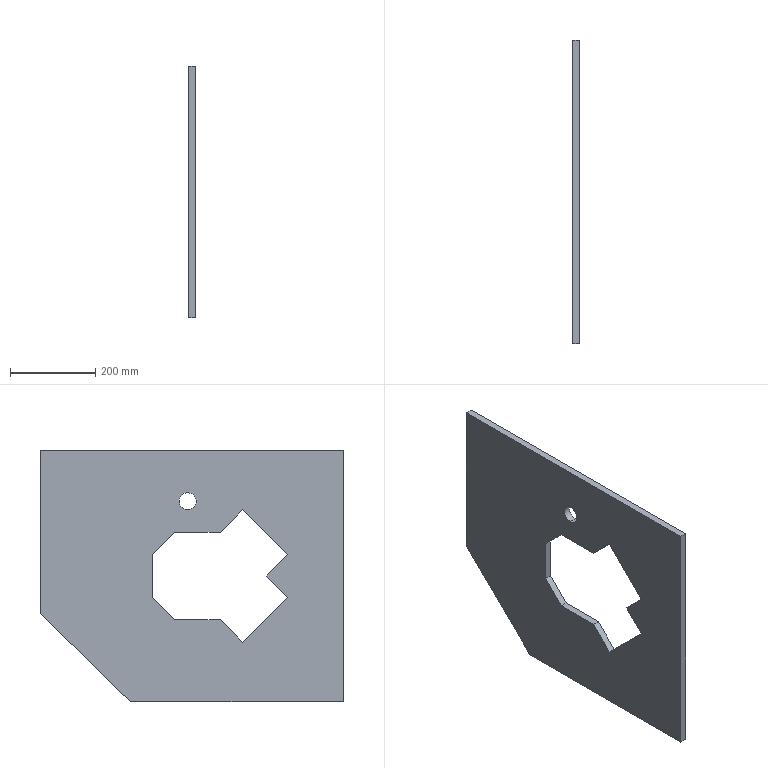Component | SolidWorks | AssemblyDriveAxis-1_16PlateModified-1 | 1 solid | 25 faces | box 16 x 710 x 590 mm | volume 5329547 mm3 | plane 23 | cylinder 2 | commonest cylinder face diameters 40 x2
build123d program:
from build123d import *

# Parameters (mm, degrees)
SKETCH1_2_W          = 590
SKETCH1_2_H          = 710
BOSS_EXTRUDE1_DEPTH  = 16
SKETCH2_R            = 20
CUT_EXTRUDE1_2_DEPTH = 16
CUT_EXTRUDE3_DEPTH   = 16
CUT_EXTRUDE1_DEPTH   = 3.5


with BuildPart() as part:
    # Sketch1_2 → Boss-Extrude1 (new body)
    with BuildSketch(Plane.XY):
        with Locations((295, 355)):
            Rectangle(SKETCH1_2_W, SKETCH1_2_H)
    extrude(amount=BOSS_EXTRUDE1_DEPTH)

    # Sketch2 → Cut-Extrude1_2 (cut)
    with BuildSketch(Plane.XY.offset(16)):
        Polygon((345, 448), (245, 448), (193, 396), (193, 289), (140, 236), (245.738, 130.262), (295, 179.524), (344.262, 130.262), (450, 236), (397, 289), (397, 396), align=None)
        with Locations((120, 365)):
            Circle(SKETCH2_R)
    extrude(amount=-CUT_EXTRUDE1_2_DEPTH, mode=Mode.SUBTRACT)

    # Sketch4 → Cut-Extrude3 (cut)
    with BuildSketch(Plane.XY.offset(16)):
        Polygon((590, 498.948), (383.169, 710), (590, 710), align=None)
    extrude(amount=-CUT_EXTRUDE3_DEPTH, mode=Mode.SUBTRACT)

    # Sketch1 → Cut-Extrude1 (cut)
    with BuildSketch(Plane.XY.offset(16)):
        Polygon((337.078, 75.224), (314.451, 97.852), (334.25, 117.651), (356.877, 95.023), align=None)
    extrude(amount=-CUT_EXTRUDE1_DEPTH, mode=Mode.SUBTRACT)


solid = part.part

# Placed as in the assembly
solid = solid.moved(Location((-141, 500, 565), (0, 90, 0)))
STEP:
#1=CARTESIAN_POINT('',(-5.551,34.055,18.307));
#2=VERTEX_POINT('',#1);
#3=CARTESIAN_POINT('',(-5.551,34.055,16.732));
#4=VERTEX_POINT('',#3);
#5=CARTESIAN_POINT('',(-5.551,34.055,17.52));
#6=DIRECTION('',(1.,-0.,0.));
#7=DIRECTION('',(0.,0.,-1.));
#8=AXIS2_PLACEMENT_3D('',#5,#6,#7);
#9=CIRCLE('',#8,0.7874);
#10=EDGE_CURVE('',#2,#4,#9,.T.);
#11=ORIENTED_EDGE('',*,*,#10,.F.);
#12=CARTESIAN_POINT('',(-4.921,34.055,18.307));
#13=VERTEX_POINT('',#12);
#14=CARTESIAN_POINT('',(-5.551,34.055,18.307));
#15=DIRECTION('',(1.,-0.,0.));
#16=VECTOR('',#15,39.37);
#17=LINE('',#14,#16);
#18=EDGE_CURVE('',#2,#13,#17,.T.);
#19=ORIENTED_EDGE('',*,*,#18,.T.);
#20=CARTESIAN_POINT('',(-4.921,34.055,16.732));
#21=VERTEX_POINT('',#20);
#22=CARTESIAN_POINT('',(-4.921,34.055,17.52));
#23=DIRECTION('',(1.,-0.,0.));
#24=DIRECTION('',(0.,0.,-1.));
#25=AXIS2_PLACEMENT_3D('',#22,#23,#24);
#26=CIRCLE('',#25,0.7874);
#27=EDGE_CURVE('',#13,#21,#26,.T.);
#28=ORIENTED_EDGE('',*,*,#27,.T.);
#29=CARTESIAN_POINT('',(-5.551,34.055,16.732));
#30=DIRECTION('',(1.,-0.,0.));
#31=VECTOR('',#30,39.37);
#32=LINE('',#29,#31);
#33=EDGE_CURVE('',#4,#21,#32,.T.);
#34=ORIENTED_EDGE('',*,*,#33,.F.);
#35=EDGE_LOOP('',(#11,#19,#28,#34));
#36=FACE_OUTER_BOUND('',#35,.T.);
#37=CARTESIAN_POINT('',(-5.551,34.055,17.52));
#38=DIRECTION('',(1.,-0.,0.));
#39=DIRECTION('',(0.,0.,-1.));
#40=AXIS2_PLACEMENT_3D('',#37,#38,#39);
#41=CYLINDRICAL_SURFACE('',#40,0.7874);
#42=ADVANCED_FACE('',(#36),#41,.F.);
#43=CARTESIAN_POINT('',(-4.921,22.647,8.973));
#44=VERTEX_POINT('',#43);
#45=CARTESIAN_POINT('',(-4.921,23.426,8.194));
#46=VERTEX_POINT('',#45);
#47=CARTESIAN_POINT('',(-4.921,23.426,8.194));
#48=DIRECTION('',(0.,0.7071,-0.7071));
#49=VECTOR('',#48,39.37);
#50=LINE('',#47,#49);
#51=EDGE_CURVE('',#44,#46,#50,.T.);
#52=ORIENTED_EDGE('',*,*,#51,.F.);
#53=CARTESIAN_POINT('',(-4.921,23.537,9.864));
#54=VERTEX_POINT('',#53);
#55=CARTESIAN_POINT('',(-4.921,22.647,8.973));
#56=DIRECTION('',(-0.,-0.7071,-0.7071));
#57=VECTOR('',#56,39.37);
#58=LINE('',#55,#57);
#59=EDGE_CURVE('',#54,#44,#58,.T.);
#60=ORIENTED_EDGE('',*,*,#59,.F.);
#61=CARTESIAN_POINT('',(-4.921,24.317,9.085));
#62=VERTEX_POINT('',#61);
#63=CARTESIAN_POINT('',(-4.921,23.537,9.864));
#64=DIRECTION('',(-0.,-0.7071,0.7071));
#65=VECTOR('',#64,39.37);
#66=LINE('',#63,#65);
#67=EDGE_CURVE('',#62,#54,#66,.T.);
#68=ORIENTED_EDGE('',*,*,#67,.F.);
#69=CARTESIAN_POINT('',(-4.921,24.317,9.085));
#70=DIRECTION('',(0.,0.7071,0.7071));
#71=VECTOR('',#70,39.37);
#72=LINE('',#69,#71);
#73=EDGE_CURVE('',#46,#62,#72,.T.);
#74=ORIENTED_EDGE('',*,*,#73,.F.);
#75=EDGE_LOOP('',(#52,#60,#68,#74));
#76=FACE_BOUND('',#75,.T.);
#77=CARTESIAN_POINT('',(-4.921,47.638,7.159));
#78=VERTEX_POINT('',#77);
#79=CARTESIAN_POINT('',(-4.921,39.329,-0.9843));
#80=VERTEX_POINT('',#79);
#81=CARTESIAN_POINT('',(-4.921,39.329,-0.9843));
#82=DIRECTION('',(-0.,-0.7142,-0.6999));
#83=VECTOR('',#82,39.37);
#84=LINE('',#81,#83);
#85=EDGE_CURVE('',#78,#80,#84,.T.);
#86=ORIENTED_EDGE('',*,*,#85,.F.);
#87=CARTESIAN_POINT('',(-4.921,47.638,22.244));
#88=VERTEX_POINT('',#87);
#89=CARTESIAN_POINT('',(-4.921,47.638,-0.9843));
#90=DIRECTION('',(-0.,0.,1.));
#91=VECTOR('',#90,39.37);
#92=LINE('',#89,#91);
#93=EDGE_CURVE('',#78,#88,#92,.T.);
#94=ORIENTED_EDGE('',*,*,#93,.T.);
#95=CARTESIAN_POINT('',(-4.921,19.685,22.244));
#96=VERTEX_POINT('',#95);
#97=CARTESIAN_POINT('',(-4.921,47.638,22.244));
#98=DIRECTION('',(-0.,-1.,-0.));
#99=VECTOR('',#98,39.37);
#100=LINE('',#97,#99);
#101=EDGE_CURVE('',#88,#96,#100,.T.);
#102=ORIENTED_EDGE('',*,*,#101,.T.);
#103=CARTESIAN_POINT('',(-4.921,19.685,-0.9843));
#104=VERTEX_POINT('',#103);
#105=CARTESIAN_POINT('',(-4.921,19.685,22.244));
#106=DIRECTION('',(0.,0.,-1.));
#107=VECTOR('',#106,39.37);
#108=LINE('',#105,#107);
#109=EDGE_CURVE('',#96,#104,#108,.T.);
#110=ORIENTED_EDGE('',*,*,#109,.T.);
#111=CARTESIAN_POINT('',(-4.921,19.685,-0.9843));
#112=DIRECTION('',(0.,1.,0.));
#113=VECTOR('',#112,39.37);
#114=LINE('',#111,#113);
#115=EDGE_CURVE('',#104,#80,#114,.T.);
#116=ORIENTED_EDGE('',*,*,#115,.T.);
#117=EDGE_LOOP('',(#86,#94,#102,#110,#116));
#118=FACE_OUTER_BOUND('',#117,.T.);
#119=CARTESIAN_POINT('',(-4.921,34.055,17.52));
#120=DIRECTION('',(1.,-0.,0.));
#121=DIRECTION('',(0.,0.,-1.));
#122=AXIS2_PLACEMENT_3D('',#119,#120,#121);
#123=CIRCLE('',#122,0.7874);
#124=EDGE_CURVE('',#21,#13,#123,.T.);
#125=ORIENTED_EDGE('',*,*,#124,.F.);
#126=ORIENTED_EDGE('',*,*,#27,.F.);
#127=EDGE_LOOP('',(#125,#126));
#128=FACE_BOUND('',#127,.T.);
#129=CARTESIAN_POINT('',(-4.921,37.323,12.598));
#130=VERTEX_POINT('',#129);
#131=CARTESIAN_POINT('',(-4.921,35.276,14.646));
#132=VERTEX_POINT('',#131);
#133=CARTESIAN_POINT('',(-4.921,23.681,26.24));
#134=DIRECTION('',(-0.,-0.7071,0.7071));
#135=VECTOR('',#134,39.37);
#136=LINE('',#133,#135);
#137=EDGE_CURVE('',#130,#132,#136,.T.);
#138=ORIENTED_EDGE('',*,*,#137,.F.);
#139=CARTESIAN_POINT('',(-4.921,37.323,8.661));
#140=VERTEX_POINT('',#139);
#141=CARTESIAN_POINT('',(-4.921,37.323,22.244));
#142=DIRECTION('',(0.,0.,-1.));
#143=VECTOR('',#142,39.37);
#144=LINE('',#141,#143);
#145=EDGE_CURVE('',#130,#140,#144,.T.);
#146=ORIENTED_EDGE('',*,*,#145,.T.);
#147=CARTESIAN_POINT('',(-4.921,35.276,6.614));
#148=VERTEX_POINT('',#147);
#149=CARTESIAN_POINT('',(-4.921,35.295,6.634));
#150=DIRECTION('',(-0.,-0.7071,-0.7071));
#151=VECTOR('',#150,39.37);
#152=LINE('',#149,#151);
#153=EDGE_CURVE('',#140,#148,#152,.T.);
#154=ORIENTED_EDGE('',*,*,#153,.T.);
#155=CARTESIAN_POINT('',(-4.921,31.063,6.614));
#156=VERTEX_POINT('',#155);
#157=CARTESIAN_POINT('',(-4.921,19.685,6.614));
#158=DIRECTION('',(-0.,-1.,0.));
#159=VECTOR('',#158,39.37);
#160=LINE('',#157,#159);
#161=EDGE_CURVE('',#148,#156,#160,.T.);
#162=ORIENTED_EDGE('',*,*,#161,.T.);
#163=CARTESIAN_POINT('',(-4.921,28.976,4.528));
#164=VERTEX_POINT('',#163);
#165=CARTESIAN_POINT('',(-4.921,33.189,8.74));
#166=DIRECTION('',(-0.,-0.7071,-0.7071));
#167=VECTOR('',#166,39.37);
#168=LINE('',#165,#167);
#169=EDGE_CURVE('',#156,#164,#168,.T.);
#170=ORIENTED_EDGE('',*,*,#169,.T.);
#171=CARTESIAN_POINT('',(-4.921,24.813,8.69));
#172=VERTEX_POINT('',#171);
#173=CARTESIAN_POINT('',(-4.921,15.472,18.031));
#174=DIRECTION('',(-0.,-0.7071,0.7071));
#175=VECTOR('',#174,39.37);
#176=LINE('',#173,#175);
#177=EDGE_CURVE('',#164,#172,#176,.T.);
#178=ORIENTED_EDGE('',*,*,#177,.T.);
#179=CARTESIAN_POINT('',(-4.921,26.753,10.63));
#180=VERTEX_POINT('',#179);
#181=CARTESIAN_POINT('',(-4.921,29.026,12.903));
#182=DIRECTION('',(0.,0.7071,0.7071));
#183=VECTOR('',#182,39.37);
#184=LINE('',#181,#183);
#185=EDGE_CURVE('',#172,#180,#184,.T.);
#186=ORIENTED_EDGE('',*,*,#185,.T.);
#187=CARTESIAN_POINT('',(-4.921,24.813,12.569));
#188=VERTEX_POINT('',#187);
#189=CARTESIAN_POINT('',(-4.921,17.412,19.971));
#190=DIRECTION('',(0.,0.7071,-0.7071));
#191=VECTOR('',#190,39.37);
#192=LINE('',#189,#191);
#193=EDGE_CURVE('',#188,#180,#192,.T.);
#194=ORIENTED_EDGE('',*,*,#193,.F.);
#195=CARTESIAN_POINT('',(-4.921,28.976,16.732));
#196=VERTEX_POINT('',#195);
#197=CARTESIAN_POINT('',(-4.921,27.087,14.843));
#198=DIRECTION('',(-0.,-0.7071,-0.7071));
#199=VECTOR('',#198,39.37);
#200=LINE('',#197,#199);
#201=EDGE_CURVE('',#196,#188,#200,.T.);
#202=ORIENTED_EDGE('',*,*,#201,.F.);
#203=CARTESIAN_POINT('',(-4.921,31.063,14.646));
#204=VERTEX_POINT('',#203);
#205=CARTESIAN_POINT('',(-4.921,21.575,24.134));
#206=DIRECTION('',(-0.,-0.7071,0.7071));
#207=VECTOR('',#206,39.37);
#208=LINE('',#205,#207);
#209=EDGE_CURVE('',#204,#196,#208,.T.);
#210=ORIENTED_EDGE('',*,*,#209,.F.);
#211=CARTESIAN_POINT('',(-4.921,19.685,14.646));
#212=DIRECTION('',(-0.,-1.,-0.));
#213=VECTOR('',#212,39.37);
#214=LINE('',#211,#213);
#215=EDGE_CURVE('',#132,#204,#214,.T.);
#216=ORIENTED_EDGE('',*,*,#215,.F.);
#217=EDGE_LOOP('',(#138,#146,#154,#162,#170,#178,#186,#194,#202,#210,#216));
#218=FACE_BOUND('',#217,.T.);
#219=CARTESIAN_POINT('',(-4.921,19.685,22.244));
#220=DIRECTION('',(1.,-0.,0.));
#221=DIRECTION('',(0.,0.,-1.));
#222=AXIS2_PLACEMENT_3D('',#219,#220,#221);
#223=PLANE('',#222);
#224=ADVANCED_FACE('',(#76,#118,#128,#218),#223,.T.);
#225=CARTESIAN_POINT('',(-5.551,34.055,17.52));
#226=DIRECTION('',(1.,-0.,0.));
#227=DIRECTION('',(0.,0.,-1.));
#228=AXIS2_PLACEMENT_3D('',#225,#226,#227);
#229=CIRCLE('',#228,0.7874);
#230=EDGE_CURVE('',#4,#2,#229,.T.);
#231=ORIENTED_EDGE('',*,*,#230,.T.);
#232=ORIENTED_EDGE('',*,*,#10,.T.);
#233=EDGE_LOOP('',(#231,#232));
#234=FACE_BOUND('',#233,.T.);
#235=CARTESIAN_POINT('',(-5.551,47.638,7.159));
#236=VERTEX_POINT('',#235);
#237=CARTESIAN_POINT('',(-5.551,47.638,22.244));
#238=VERTEX_POINT('',#237);
#239=CARTESIAN_POINT('',(-5.551,47.638,-0.9843));
#240=DIRECTION('',(-0.,0.,1.));
#241=VECTOR('',#240,39.37);
#242=LINE('',#239,#241);
#243=EDGE_CURVE('',#236,#238,#242,.T.);
#244=ORIENTED_EDGE('',*,*,#243,.F.);
#245=CARTESIAN_POINT('',(-5.551,39.329,-0.9843));
#246=VERTEX_POINT('',#245);
#247=CARTESIAN_POINT('',(-5.551,39.329,-0.9843));
#248=DIRECTION('',(-0.,-0.7142,-0.6999));
#249=VECTOR('',#248,39.37);
#250=LINE('',#247,#249);
#251=EDGE_CURVE('',#236,#246,#250,.T.);
#252=ORIENTED_EDGE('',*,*,#251,.T.);
#253=CARTESIAN_POINT('',(-5.551,19.685,-0.9843));
#254=VERTEX_POINT('',#253);
#255=CARTESIAN_POINT('',(-5.551,19.685,-0.9843));
#256=DIRECTION('',(0.,1.,0.));
#257=VECTOR('',#256,39.37);
#258=LINE('',#255,#257);
#259=EDGE_CURVE('',#254,#246,#258,.T.);
#260=ORIENTED_EDGE('',*,*,#259,.F.);
#261=CARTESIAN_POINT('',(-5.551,19.685,22.244));
#262=VERTEX_POINT('',#261);
#263=CARTESIAN_POINT('',(-5.551,19.685,22.244));
#264=DIRECTION('',(0.,0.,-1.));
#265=VECTOR('',#264,39.37);
#266=LINE('',#263,#265);
#267=EDGE_CURVE('',#262,#254,#266,.T.);
#268=ORIENTED_EDGE('',*,*,#267,.F.);
#269=CARTESIAN_POINT('',(-5.551,47.638,22.244));
#270=DIRECTION('',(-0.,-1.,-0.));
#271=VECTOR('',#270,39.37);
#272=LINE('',#269,#271);
#273=EDGE_CURVE('',#238,#262,#272,.T.);
#274=ORIENTED_EDGE('',*,*,#273,.F.);
#275=EDGE_LOOP('',(#244,#252,#260,#268,#274));
#276=FACE_OUTER_BOUND('',#275,.T.);
#277=CARTESIAN_POINT('',(-5.551,37.323,12.598));
#278=VERTEX_POINT('',#277);
#279=CARTESIAN_POINT('',(-5.551,37.323,8.661));
#280=VERTEX_POINT('',#279);
#281=CARTESIAN_POINT('',(-5.551,37.323,22.244));
#282=DIRECTION('',(0.,0.,-1.));
#283=VECTOR('',#282,39.37);
#284=LINE('',#281,#283);
#285=EDGE_CURVE('',#278,#280,#284,.T.);
#286=ORIENTED_EDGE('',*,*,#285,.F.);
#287=CARTESIAN_POINT('',(-5.551,35.276,14.646));
#288=VERTEX_POINT('',#287);
#289=CARTESIAN_POINT('',(-5.551,23.681,26.24));
#290=DIRECTION('',(-0.,-0.7071,0.7071));
#291=VECTOR('',#290,39.37);
#292=LINE('',#289,#291);
#293=EDGE_CURVE('',#278,#288,#292,.T.);
#294=ORIENTED_EDGE('',*,*,#293,.T.);
#295=CARTESIAN_POINT('',(-5.551,31.063,14.646));
#296=VERTEX_POINT('',#295);
#297=CARTESIAN_POINT('',(-5.551,19.685,14.646));
#298=DIRECTION('',(-0.,-1.,-0.));
#299=VECTOR('',#298,39.37);
#300=LINE('',#297,#299);
#301=EDGE_CURVE('',#288,#296,#300,.T.);
#302=ORIENTED_EDGE('',*,*,#301,.T.);
#303=CARTESIAN_POINT('',(-5.551,28.976,16.732));
#304=VERTEX_POINT('',#303);
#305=CARTESIAN_POINT('',(-5.551,21.575,24.134));
#306=DIRECTION('',(-0.,-0.7071,0.7071));
#307=VECTOR('',#306,39.37);
#308=LINE('',#305,#307);
#309=EDGE_CURVE('',#296,#304,#308,.T.);
#310=ORIENTED_EDGE('',*,*,#309,.T.);
#311=CARTESIAN_POINT('',(-5.551,24.813,12.569));
#312=VERTEX_POINT('',#311);
#313=CARTESIAN_POINT('',(-5.551,27.087,14.843));
#314=DIRECTION('',(-0.,-0.7071,-0.7071));
#315=VECTOR('',#314,39.37);
#316=LINE('',#313,#315);
#317=EDGE_CURVE('',#304,#312,#316,.T.);
#318=ORIENTED_EDGE('',*,*,#317,.T.);
#319=CARTESIAN_POINT('',(-5.551,26.753,10.63));
#320=VERTEX_POINT('',#319);
#321=CARTESIAN_POINT('',(-5.551,17.412,19.971));
#322=DIRECTION('',(0.,0.7071,-0.7071));
#323=VECTOR('',#322,39.37);
#324=LINE('',#321,#323);
#325=EDGE_CURVE('',#312,#320,#324,.T.);
#326=ORIENTED_EDGE('',*,*,#325,.T.);
#327=CARTESIAN_POINT('',(-5.551,24.813,8.69));
#328=VERTEX_POINT('',#327);
#329=CARTESIAN_POINT('',(-5.551,29.026,12.903));
#330=DIRECTION('',(0.,0.7071,0.7071));
#331=VECTOR('',#330,39.37);
#332=LINE('',#329,#331);
#333=EDGE_CURVE('',#328,#320,#332,.T.);
#334=ORIENTED_EDGE('',*,*,#333,.F.);
#335=CARTESIAN_POINT('',(-5.551,28.976,4.528));
#336=VERTEX_POINT('',#335);
#337=CARTESIAN_POINT('',(-5.551,15.472,18.031));
#338=DIRECTION('',(-0.,-0.7071,0.7071));
#339=VECTOR('',#338,39.37);
#340=LINE('',#337,#339);
#341=EDGE_CURVE('',#336,#328,#340,.T.);
#342=ORIENTED_EDGE('',*,*,#341,.F.);
#343=CARTESIAN_POINT('',(-5.551,31.063,6.614));
#344=VERTEX_POINT('',#343);
#345=CARTESIAN_POINT('',(-5.551,33.189,8.74));
#346=DIRECTION('',(-0.,-0.7071,-0.7071));
#347=VECTOR('',#346,39.37);
#348=LINE('',#345,#347);
#349=EDGE_CURVE('',#344,#336,#348,.T.);
#350=ORIENTED_EDGE('',*,*,#349,.F.);
#351=CARTESIAN_POINT('',(-5.551,35.276,6.614));
#352=VERTEX_POINT('',#351);
#353=CARTESIAN_POINT('',(-5.551,19.685,6.614));
#354=DIRECTION('',(-0.,-1.,0.));
#355=VECTOR('',#354,39.37);
#356=LINE('',#353,#355);
#357=EDGE_CURVE('',#352,#344,#356,.T.);
#358=ORIENTED_EDGE('',*,*,#357,.F.);
#359=CARTESIAN_POINT('',(-5.551,35.295,6.634));
#360=DIRECTION('',(-0.,-0.7071,-0.7071));
#361=VECTOR('',#360,39.37);
#362=LINE('',#359,#361);
#363=EDGE_CURVE('',#280,#352,#362,.T.);
#364=ORIENTED_EDGE('',*,*,#363,.F.);
#365=EDGE_LOOP('',(#286,#294,#302,#310,#318,#326,#334,#342,#350,#358,#364));
#366=FACE_BOUND('',#365,.T.);
#367=CARTESIAN_POINT('',(-5.551,19.685,22.244));
#368=DIRECTION('',(1.,-0.,0.));
#369=DIRECTION('',(0.,0.,-1.));
#370=AXIS2_PLACEMENT_3D('',#367,#368,#369);
#371=PLANE('',#370);
#372=ADVANCED_FACE('',(#234,#276,#366),#371,.F.);
#373=ORIENTED_EDGE('',*,*,#273,.T.);
#374=CARTESIAN_POINT('',(-4.921,19.685,22.244));
#375=DIRECTION('',(-1.,0.,-0.));
#376=VECTOR('',#375,39.37);
#377=LINE('',#374,#376);
#378=EDGE_CURVE('',#96,#262,#377,.T.);
#379=ORIENTED_EDGE('',*,*,#378,.F.);
#380=ORIENTED_EDGE('',*,*,#101,.F.);
#381=CARTESIAN_POINT('',(-4.921,47.638,22.244));
#382=DIRECTION('',(-1.,0.,-0.));
#383=VECTOR('',#382,39.37);
#384=LINE('',#381,#383);
#385=EDGE_CURVE('',#88,#238,#384,.T.);
#386=ORIENTED_EDGE('',*,*,#385,.T.);
#387=EDGE_LOOP('',(#373,#379,#380,#386));
#388=FACE_OUTER_BOUND('',#387,.T.);
#389=CARTESIAN_POINT('',(-4.921,47.638,22.244));
#390=DIRECTION('',(0.,0.,-1.));
#391=DIRECTION('',(0.,1.,0.));
#392=AXIS2_PLACEMENT_3D('',#389,#390,#391);
#393=PLANE('',#392);
#394=ADVANCED_FACE('',(#388),#393,.F.);
#395=ORIENTED_EDGE('',*,*,#267,.T.);
#396=CARTESIAN_POINT('',(-4.921,19.685,-0.9843));
#397=DIRECTION('',(-1.,0.,-0.));
#398=VECTOR('',#397,39.37);
#399=LINE('',#396,#398);
#400=EDGE_CURVE('',#104,#254,#399,.T.);
#401=ORIENTED_EDGE('',*,*,#400,.F.);
#402=ORIENTED_EDGE('',*,*,#109,.F.);
#403=ORIENTED_EDGE('',*,*,#378,.T.);
#404=EDGE_LOOP('',(#395,#401,#402,#403));
#405=FACE_OUTER_BOUND('',#404,.T.);
#406=CARTESIAN_POINT('',(-4.921,19.685,22.244));
#407=DIRECTION('',(0.,1.,0.));
#408=DIRECTION('',(1.,-0.,0.));
#409=AXIS2_PLACEMENT_3D('',#406,#407,#408);
#410=PLANE('',#409);
#411=ADVANCED_FACE('',(#405),#410,.F.);
#412=ORIENTED_EDGE('',*,*,#259,.T.);
#413=CARTESIAN_POINT('',(-5.551,39.329,-0.9843));
#414=DIRECTION('',(1.,-0.,0.));
#415=VECTOR('',#414,39.37);
#416=LINE('',#413,#415);
#417=EDGE_CURVE('',#246,#80,#416,.T.);
#418=ORIENTED_EDGE('',*,*,#417,.T.);
#419=ORIENTED_EDGE('',*,*,#115,.F.);
#420=ORIENTED_EDGE('',*,*,#400,.T.);
#421=EDGE_LOOP('',(#412,#418,#419,#420));
#422=FACE_OUTER_BOUND('',#421,.T.);
#423=CARTESIAN_POINT('',(-4.921,19.685,-0.9843));
#424=DIRECTION('',(-0.,0.,1.));
#425=DIRECTION('',(1.,-0.,0.));
#426=AXIS2_PLACEMENT_3D('',#423,#424,#425);
#427=PLANE('',#426);
#428=ADVANCED_FACE('',(#422),#427,.F.);
#429=ORIENTED_EDGE('',*,*,#93,.F.);
#430=CARTESIAN_POINT('',(-5.551,47.638,7.159));
#431=DIRECTION('',(1.,-0.,0.));
#432=VECTOR('',#431,39.37);
#433=LINE('',#430,#432);
#434=EDGE_CURVE('',#236,#78,#433,.T.);
#435=ORIENTED_EDGE('',*,*,#434,.F.);
#436=ORIENTED_EDGE('',*,*,#243,.T.);
#437=ORIENTED_EDGE('',*,*,#385,.F.);
#438=EDGE_LOOP('',(#429,#435,#436,#437));
#439=FACE_OUTER_BOUND('',#438,.T.);
#440=CARTESIAN_POINT('',(-4.921,47.638,-0.9843));
#441=DIRECTION('',(-0.,-1.,-0.));
#442=DIRECTION('',(-1.,0.,-0.));
#443=AXIS2_PLACEMENT_3D('',#440,#441,#442);
#444=PLANE('',#443);
#445=ADVANCED_FACE('',(#439),#444,.F.);
#446=ORIENTED_EDGE('',*,*,#145,.F.);
#447=CARTESIAN_POINT('',(-5.551,37.323,12.598));
#448=DIRECTION('',(1.,-0.,0.));
#449=VECTOR('',#448,39.37);
#450=LINE('',#447,#449);
#451=EDGE_CURVE('',#278,#130,#450,.T.);
#452=ORIENTED_EDGE('',*,*,#451,.F.);
#453=ORIENTED_EDGE('',*,*,#285,.T.);
#454=CARTESIAN_POINT('',(-5.551,37.323,8.661));
#455=DIRECTION('',(1.,-0.,0.));
#456=VECTOR('',#455,39.37);
#457=LINE('',#454,#456);
#458=EDGE_CURVE('',#280,#140,#457,.T.);
#459=ORIENTED_EDGE('',*,*,#458,.T.);
#460=EDGE_LOOP('',(#446,#452,#453,#459));
#461=FACE_OUTER_BOUND('',#460,.T.);
#462=CARTESIAN_POINT('',(-5.551,37.323,22.244));
#463=DIRECTION('',(-0.,-1.,-0.));
#464=DIRECTION('',(-1.,0.,-0.));
#465=AXIS2_PLACEMENT_3D('',#462,#463,#464);
#466=PLANE('',#465);
#467=ADVANCED_FACE('',(#461),#466,.T.);
#468=ORIENTED_EDGE('',*,*,#153,.F.);
#469=ORIENTED_EDGE('',*,*,#458,.F.);
#470=ORIENTED_EDGE('',*,*,#363,.T.);
#471=CARTESIAN_POINT('',(-5.551,35.276,6.614));
#472=DIRECTION('',(1.,-0.,0.));
#473=VECTOR('',#472,39.37);
#474=LINE('',#471,#473);
#475=EDGE_CURVE('',#352,#148,#474,.T.);
#476=ORIENTED_EDGE('',*,*,#475,.T.);
#477=EDGE_LOOP('',(#468,#469,#470,#476));
#478=FACE_OUTER_BOUND('',#477,.T.);
#479=CARTESIAN_POINT('',(-5.551,35.295,6.634));
#480=DIRECTION('',(-0.,-0.7071,0.7071));
#481=DIRECTION('',(-0.,-0.7071,-0.7071));
#482=AXIS2_PLACEMENT_3D('',#479,#480,#481);
#483=PLANE('',#482);
#484=ADVANCED_FACE('',(#478),#483,.T.);
#485=ORIENTED_EDGE('',*,*,#161,.F.);
#486=ORIENTED_EDGE('',*,*,#475,.F.);
#487=ORIENTED_EDGE('',*,*,#357,.T.);
#488=CARTESIAN_POINT('',(-5.551,31.063,6.614));
#489=DIRECTION('',(1.,-0.,0.));
#490=VECTOR('',#489,39.37);
#491=LINE('',#488,#490);
#492=EDGE_CURVE('',#344,#156,#491,.T.);
#493=ORIENTED_EDGE('',*,*,#492,.T.);
#494=EDGE_LOOP('',(#485,#486,#487,#493));
#495=FACE_OUTER_BOUND('',#494,.T.);
#496=CARTESIAN_POINT('',(-5.551,19.685,6.614));
#497=DIRECTION('',(-0.,0.,1.));
#498=DIRECTION('',(1.,-0.,0.));
#499=AXIS2_PLACEMENT_3D('',#496,#497,#498);
#500=PLANE('',#499);
#501=ADVANCED_FACE('',(#495),#500,.T.);
#502=ORIENTED_EDGE('',*,*,#169,.F.);
#503=ORIENTED_EDGE('',*,*,#492,.F.);
#504=ORIENTED_EDGE('',*,*,#349,.T.);
#505=CARTESIAN_POINT('',(-5.551,28.976,4.528));
#506=DIRECTION('',(1.,-0.,0.));
#507=VECTOR('',#506,39.37);
#508=LINE('',#505,#507);
#509=EDGE_CURVE('',#336,#164,#508,.T.);
#510=ORIENTED_EDGE('',*,*,#509,.T.);
#511=EDGE_LOOP('',(#502,#503,#504,#510));
#512=FACE_OUTER_BOUND('',#511,.T.);
#513=CARTESIAN_POINT('',(-5.551,33.189,8.74));
#514=DIRECTION('',(-0.,-0.7071,0.7071));
#515=DIRECTION('',(-0.,-0.7071,-0.7071));
#516=AXIS2_PLACEMENT_3D('',#513,#514,#515);
#517=PLANE('',#516);
#518=ADVANCED_FACE('',(#512),#517,.T.);
#519=ORIENTED_EDGE('',*,*,#177,.F.);
#520=ORIENTED_EDGE('',*,*,#509,.F.);
#521=ORIENTED_EDGE('',*,*,#341,.T.);
#522=CARTESIAN_POINT('',(-5.551,24.813,8.69));
#523=DIRECTION('',(1.,-0.,0.));
#524=VECTOR('',#523,39.37);
#525=LINE('',#522,#524);
#526=EDGE_CURVE('',#328,#172,#525,.T.);
#527=ORIENTED_EDGE('',*,*,#526,.T.);
#528=EDGE_LOOP('',(#519,#520,#521,#527));
#529=FACE_OUTER_BOUND('',#528,.T.);
#530=CARTESIAN_POINT('',(-5.551,15.472,18.031));
#531=DIRECTION('',(0.,0.7071,0.7071));
#532=DIRECTION('',(-0.,-0.7071,0.7071));
#533=AXIS2_PLACEMENT_3D('',#530,#531,#532);
#534=PLANE('',#533);
#535=ADVANCED_FACE('',(#529),#534,.T.);
#536=ORIENTED_EDGE('',*,*,#185,.F.);
#537=ORIENTED_EDGE('',*,*,#526,.F.);
#538=ORIENTED_EDGE('',*,*,#333,.T.);
#539=CARTESIAN_POINT('',(-5.551,26.753,10.63));
#540=DIRECTION('',(1.,-0.,0.));
#541=VECTOR('',#540,39.37);
#542=LINE('',#539,#541);
#543=EDGE_CURVE('',#320,#180,#542,.T.);
#544=ORIENTED_EDGE('',*,*,#543,.T.);
#545=EDGE_LOOP('',(#536,#537,#538,#544));
#546=FACE_OUTER_BOUND('',#545,.T.);
#547=CARTESIAN_POINT('',(-5.551,29.026,12.903));
#548=DIRECTION('',(0.,0.7071,-0.7071));
#549=DIRECTION('',(0.,0.7071,0.7071));
#550=AXIS2_PLACEMENT_3D('',#547,#548,#549);
#551=PLANE('',#550);
#552=ADVANCED_FACE('',(#546),#551,.T.);
#553=ORIENTED_EDGE('',*,*,#193,.T.);
#554=ORIENTED_EDGE('',*,*,#543,.F.);
#555=ORIENTED_EDGE('',*,*,#325,.F.);
#556=CARTESIAN_POINT('',(-5.551,24.813,12.569));
#557=DIRECTION('',(1.,-0.,0.));
#558=VECTOR('',#557,39.37);
#559=LINE('',#556,#558);
#560=EDGE_CURVE('',#312,#188,#559,.T.);
#561=ORIENTED_EDGE('',*,*,#560,.T.);
#562=EDGE_LOOP('',(#553,#554,#555,#561));
#563=FACE_OUTER_BOUND('',#562,.T.);
#564=CARTESIAN_POINT('',(-5.551,17.412,19.971));
#565=DIRECTION('',(-0.,-0.7071,-0.7071));
#566=DIRECTION('',(0.,0.7071,-0.7071));
#567=AXIS2_PLACEMENT_3D('',#564,#565,#566);
#568=PLANE('',#567);
#569=ADVANCED_FACE('',(#563),#568,.F.);
#570=ORIENTED_EDGE('',*,*,#201,.T.);
#571=ORIENTED_EDGE('',*,*,#560,.F.);
#572=ORIENTED_EDGE('',*,*,#317,.F.);
#573=CARTESIAN_POINT('',(-5.551,28.976,16.732));
#574=DIRECTION('',(1.,-0.,0.));
#575=VECTOR('',#574,39.37);
#576=LINE('',#573,#575);
#577=EDGE_CURVE('',#304,#196,#576,.T.);
#578=ORIENTED_EDGE('',*,*,#577,.T.);
#579=EDGE_LOOP('',(#570,#571,#572,#578));
#580=FACE_OUTER_BOUND('',#579,.T.);
#581=CARTESIAN_POINT('',(-5.551,27.087,14.843));
#582=DIRECTION('',(-0.,-0.7071,0.7071));
#583=DIRECTION('',(-0.,-0.7071,-0.7071));
#584=AXIS2_PLACEMENT_3D('',#581,#582,#583);
#585=PLANE('',#584);
#586=ADVANCED_FACE('',(#580),#585,.F.);
#587=ORIENTED_EDGE('',*,*,#209,.T.);
#588=ORIENTED_EDGE('',*,*,#577,.F.);
#589=ORIENTED_EDGE('',*,*,#309,.F.);
#590=CARTESIAN_POINT('',(-5.551,31.063,14.646));
#591=DIRECTION('',(1.,-0.,0.));
#592=VECTOR('',#591,39.37);
#593=LINE('',#590,#592);
#594=EDGE_CURVE('',#296,#204,#593,.T.);
#595=ORIENTED_EDGE('',*,*,#594,.T.);
#596=EDGE_LOOP('',(#587,#588,#589,#595));
#597=FACE_OUTER_BOUND('',#596,.T.);
#598=CARTESIAN_POINT('',(-5.551,21.575,24.134));
#599=DIRECTION('',(0.,0.7071,0.7071));
#600=DIRECTION('',(-0.,-0.7071,0.7071));
#601=AXIS2_PLACEMENT_3D('',#598,#599,#600);
#602=PLANE('',#601);
#603=ADVANCED_FACE('',(#597),#602,.F.);
#604=ORIENTED_EDGE('',*,*,#215,.T.);
#605=ORIENTED_EDGE('',*,*,#594,.F.);
#606=ORIENTED_EDGE('',*,*,#301,.F.);
#607=CARTESIAN_POINT('',(-5.551,35.276,14.646));
#608=DIRECTION('',(1.,-0.,0.));
#609=VECTOR('',#608,39.37);
#610=LINE('',#607,#609);
#611=EDGE_CURVE('',#288,#132,#610,.T.);
#612=ORIENTED_EDGE('',*,*,#611,.T.);
#613=EDGE_LOOP('',(#604,#605,#606,#612));
#614=FACE_OUTER_BOUND('',#613,.T.);
#615=CARTESIAN_POINT('',(-5.551,19.685,14.646));
#616=DIRECTION('',(-0.,-0.,1.));
#617=DIRECTION('',(-0.,-1.,-0.));
#618=AXIS2_PLACEMENT_3D('',#615,#616,#617);
#619=PLANE('',#618);
#620=ADVANCED_FACE('',(#614),#619,.F.);
#621=ORIENTED_EDGE('',*,*,#137,.T.);
#622=ORIENTED_EDGE('',*,*,#611,.F.);
#623=ORIENTED_EDGE('',*,*,#293,.F.);
#624=ORIENTED_EDGE('',*,*,#451,.T.);
#625=EDGE_LOOP('',(#621,#622,#623,#624));
#626=FACE_OUTER_BOUND('',#625,.T.);
#627=CARTESIAN_POINT('',(-5.551,23.681,26.24));
#628=DIRECTION('',(0.,0.7071,0.7071));
#629=DIRECTION('',(-0.,-0.7071,0.7071));
#630=AXIS2_PLACEMENT_3D('',#627,#628,#629);
#631=PLANE('',#630);
#632=ADVANCED_FACE('',(#626),#631,.F.);
#633=ORIENTED_EDGE('',*,*,#18,.F.);
#634=ORIENTED_EDGE('',*,*,#230,.F.);
#635=ORIENTED_EDGE('',*,*,#33,.T.);
#636=ORIENTED_EDGE('',*,*,#124,.T.);
#637=EDGE_LOOP('',(#633,#634,#635,#636));
#638=FACE_OUTER_BOUND('',#637,.T.);
#639=CARTESIAN_POINT('',(-5.551,34.055,17.52));
#640=DIRECTION('',(1.,-0.,0.));
#641=DIRECTION('',(0.,0.,-1.));
#642=AXIS2_PLACEMENT_3D('',#639,#640,#641);
#643=CYLINDRICAL_SURFACE('',#642,0.7874);
#644=ADVANCED_FACE('',(#638),#643,.F.);
#645=ORIENTED_EDGE('',*,*,#85,.T.);
#646=ORIENTED_EDGE('',*,*,#417,.F.);
#647=ORIENTED_EDGE('',*,*,#251,.F.);
#648=ORIENTED_EDGE('',*,*,#434,.T.);
#649=EDGE_LOOP('',(#645,#646,#647,#648));
#650=FACE_OUTER_BOUND('',#649,.T.);
#651=CARTESIAN_POINT('',(-5.551,39.329,-0.9843));
#652=DIRECTION('',(-0.,-0.6999,0.7142));
#653=DIRECTION('',(-0.,-0.7142,-0.6999));
#654=AXIS2_PLACEMENT_3D('',#651,#652,#653);
#655=PLANE('',#654);
#656=ADVANCED_FACE('',(#650),#655,.F.);
#657=ORIENTED_EDGE('',*,*,#51,.T.);
#658=CARTESIAN_POINT('',(-5.059,23.426,8.194));
#659=VERTEX_POINT('',#658);
#660=CARTESIAN_POINT('',(-5.059,23.426,8.194));
#661=DIRECTION('',(1.,-0.,0.));
#662=VECTOR('',#661,39.37);
#663=LINE('',#660,#662);
#664=EDGE_CURVE('',#659,#46,#663,.T.);
#665=ORIENTED_EDGE('',*,*,#664,.F.);
#666=CARTESIAN_POINT('',(-5.059,22.647,8.973));
#667=VERTEX_POINT('',#666);
#668=CARTESIAN_POINT('',(-5.059,23.426,8.194));
#669=DIRECTION('',(0.,0.7071,-0.7071));
#670=VECTOR('',#669,39.37);
#671=LINE('',#668,#670);
#672=EDGE_CURVE('',#667,#659,#671,.T.);
#673=ORIENTED_EDGE('',*,*,#672,.F.);
#674=CARTESIAN_POINT('',(-5.059,22.647,8.973));
#675=DIRECTION('',(1.,-0.,0.));
#676=VECTOR('',#675,39.37);
#677=LINE('',#674,#676);
#678=EDGE_CURVE('',#667,#44,#677,.T.);
#679=ORIENTED_EDGE('',*,*,#678,.T.);
#680=EDGE_LOOP('',(#657,#665,#673,#679));
#681=FACE_OUTER_BOUND('',#680,.T.);
#682=CARTESIAN_POINT('',(-5.059,23.426,8.194));
#683=DIRECTION('',(-0.,-0.7071,-0.7071));
#684=DIRECTION('',(0.,0.7071,-0.7071));
#685=AXIS2_PLACEMENT_3D('',#682,#683,#684);
#686=PLANE('',#685);
#687=ADVANCED_FACE('',(#681),#686,.F.);
#688=ORIENTED_EDGE('',*,*,#59,.T.);
#689=ORIENTED_EDGE('',*,*,#678,.F.);
#690=CARTESIAN_POINT('',(-5.059,23.537,9.864));
#691=VERTEX_POINT('',#690);
#692=CARTESIAN_POINT('',(-5.059,22.647,8.973));
#693=DIRECTION('',(-0.,-0.7071,-0.7071));
#694=VECTOR('',#693,39.37);
#695=LINE('',#692,#694);
#696=EDGE_CURVE('',#691,#667,#695,.T.);
#697=ORIENTED_EDGE('',*,*,#696,.F.);
#698=CARTESIAN_POINT('',(-5.059,23.537,9.864));
#699=DIRECTION('',(1.,-0.,0.));
#700=VECTOR('',#699,39.37);
#701=LINE('',#698,#700);
#702=EDGE_CURVE('',#691,#54,#701,.T.);
#703=ORIENTED_EDGE('',*,*,#702,.T.);
#704=EDGE_LOOP('',(#688,#689,#697,#703));
#705=FACE_OUTER_BOUND('',#704,.T.);
#706=CARTESIAN_POINT('',(-5.059,22.647,8.973));
#707=DIRECTION('',(-0.,-0.7071,0.7071));
#708=DIRECTION('',(-0.,-0.7071,-0.7071));
#709=AXIS2_PLACEMENT_3D('',#706,#707,#708);
#710=PLANE('',#709);
#711=ADVANCED_FACE('',(#705),#710,.F.);
#712=ORIENTED_EDGE('',*,*,#67,.T.);
#713=ORIENTED_EDGE('',*,*,#702,.F.);
#714=CARTESIAN_POINT('',(-5.059,24.317,9.085));
#715=VERTEX_POINT('',#714);
#716=CARTESIAN_POINT('',(-5.059,23.537,9.864));
#717=DIRECTION('',(-0.,-0.7071,0.7071));
#718=VECTOR('',#717,39.37);
#719=LINE('',#716,#718);
#720=EDGE_CURVE('',#715,#691,#719,.T.);
#721=ORIENTED_EDGE('',*,*,#720,.F.);
#722=CARTESIAN_POINT('',(-5.059,24.317,9.085));
#723=DIRECTION('',(1.,-0.,0.));
#724=VECTOR('',#723,39.37);
#725=LINE('',#722,#724);
#726=EDGE_CURVE('',#715,#62,#725,.T.);
#727=ORIENTED_EDGE('',*,*,#726,.T.);
#728=EDGE_LOOP('',(#712,#713,#721,#727));
#729=FACE_OUTER_BOUND('',#728,.T.);
#730=CARTESIAN_POINT('',(-5.059,23.537,9.864));
#731=DIRECTION('',(0.,0.7071,0.7071));
#732=DIRECTION('',(-0.,-0.7071,0.7071));
#733=AXIS2_PLACEMENT_3D('',#730,#731,#732);
#734=PLANE('',#733);
#735=ADVANCED_FACE('',(#729),#734,.F.);
#736=ORIENTED_EDGE('',*,*,#73,.T.);
#737=ORIENTED_EDGE('',*,*,#726,.F.);
#738=CARTESIAN_POINT('',(-5.059,24.317,9.085));
#739=DIRECTION('',(0.,0.7071,0.7071));
#740=VECTOR('',#739,39.37);
#741=LINE('',#738,#740);
#742=EDGE_CURVE('',#659,#715,#741,.T.);
#743=ORIENTED_EDGE('',*,*,#742,.F.);
#744=ORIENTED_EDGE('',*,*,#664,.T.);
#745=EDGE_LOOP('',(#736,#737,#743,#744));
#746=FACE_OUTER_BOUND('',#745,.T.);
#747=CARTESIAN_POINT('',(-5.059,24.317,9.085));
#748=DIRECTION('',(0.,0.7071,-0.7071));
#749=DIRECTION('',(0.,0.7071,0.7071));
#750=AXIS2_PLACEMENT_3D('',#747,#748,#749);
#751=PLANE('',#750);
#752=ADVANCED_FACE('',(#746),#751,.F.);
#753=ORIENTED_EDGE('',*,*,#672,.T.);
#754=ORIENTED_EDGE('',*,*,#742,.T.);
#755=ORIENTED_EDGE('',*,*,#720,.T.);
#756=ORIENTED_EDGE('',*,*,#696,.T.);
#757=EDGE_LOOP('',(#753,#754,#755,#756));
#758=FACE_OUTER_BOUND('',#757,.T.);
#759=CARTESIAN_POINT('',(-5.059,19.685,22.244));
#760=DIRECTION('',(-1.,0.,-0.));
#761=DIRECTION('',(-0.,0.,1.));
#762=AXIS2_PLACEMENT_3D('',#759,#760,#761);
#763=PLANE('',#762);
#764=ADVANCED_FACE('',(#758),#763,.F.);
#765=CLOSED_SHELL('',(#42,#224,#372,#394,#411,#428,#445,#467,#484,#501,#518,#535,#552,#569,#586,#603,#620,#632,#644,#656,#687,#711,#735,#752,#764));
#766=MANIFOLD_SOLID_BREP('',#765);
#767=CARTESIAN_POINT('',(0.,0.,0.));
#768=DIRECTION('',(0.,0.,1.));
#769=DIRECTION('',(1.,0.,0.));
#770=AXIS2_PLACEMENT_3D('',#767,#768,#769);
#771=(LENGTH_UNIT()NAMED_UNIT(*)SI_UNIT($,.METRE.));
#772=LENGTH_MEASURE_WITH_UNIT(LENGTH_MEASURE(0.0254),#771);
#773=DIMENSIONAL_EXPONENTS(1.,0.,0.,0.,0.,0.,0.);
#774=(CONVERSION_BASED_UNIT('',#772)LENGTH_UNIT()NAMED_UNIT(#773));
#775=UNCERTAINTY_MEASURE_WITH_UNIT(LENGTH_MEASURE(0.00001),#774,'','');
#776=(NAMED_UNIT(*)PLANE_ANGLE_UNIT()SI_UNIT($,.RADIAN.));
#777=(NAMED_UNIT(*)SI_UNIT($,.STERADIAN.)SOLID_ANGLE_UNIT());
#778=(GEOMETRIC_REPRESENTATION_CONTEXT(3)GLOBAL_UNCERTAINTY_ASSIGNED_CONTEXT((#775))GLOBAL_UNIT_ASSIGNED_CONTEXT((#774,#776,#777))REPRESENTATION_CONTEXT('',''));
#779=ADVANCED_BREP_SHAPE_REPRESENTATION('',(#766,#770),#778);
#780=COLOUR_RGB('',0.7922,0.8196,0.9333);
#781=FILL_AREA_STYLE_COLOUR('',#780);
#782=FILL_AREA_STYLE('',(#781));
#783=SURFACE_STYLE_FILL_AREA(#782);
#784=SURFACE_SIDE_STYLE('',(#783));
#785=SURFACE_STYLE_USAGE(.BOTH.,#784);
#786=PRESENTATION_STYLE_ASSIGNMENT((#785));
#787=STYLED_ITEM('',(#786),#766);
#788=PRESENTATION_LAYER_ASSIGNMENT('','',(#787));
#789=(LENGTH_UNIT()NAMED_UNIT(*)SI_UNIT($,.METRE.));
#790=LENGTH_MEASURE_WITH_UNIT(LENGTH_MEASURE(0.0254),#789);
#791=DIMENSIONAL_EXPONENTS(1.,0.,0.,0.,0.,0.,0.);
#792=(CONVERSION_BASED_UNIT('',#790)LENGTH_UNIT()NAMED_UNIT(#791));
#793=UNCERTAINTY_MEASURE_WITH_UNIT(LENGTH_MEASURE(0.00001),#792,'','');
#794=(NAMED_UNIT(*)PLANE_ANGLE_UNIT()SI_UNIT($,.RADIAN.));
#795=(NAMED_UNIT(*)SI_UNIT($,.STERADIAN.)SOLID_ANGLE_UNIT());
#796=(GEOMETRIC_REPRESENTATION_CONTEXT(3)GLOBAL_UNCERTAINTY_ASSIGNED_CONTEXT((#793))GLOBAL_UNIT_ASSIGNED_CONTEXT((#792,#794,#795))REPRESENTATION_CONTEXT('',''));
#797=MECHANICAL_DESIGN_GEOMETRIC_PRESENTATION_REPRESENTATION('',(#787),#796);